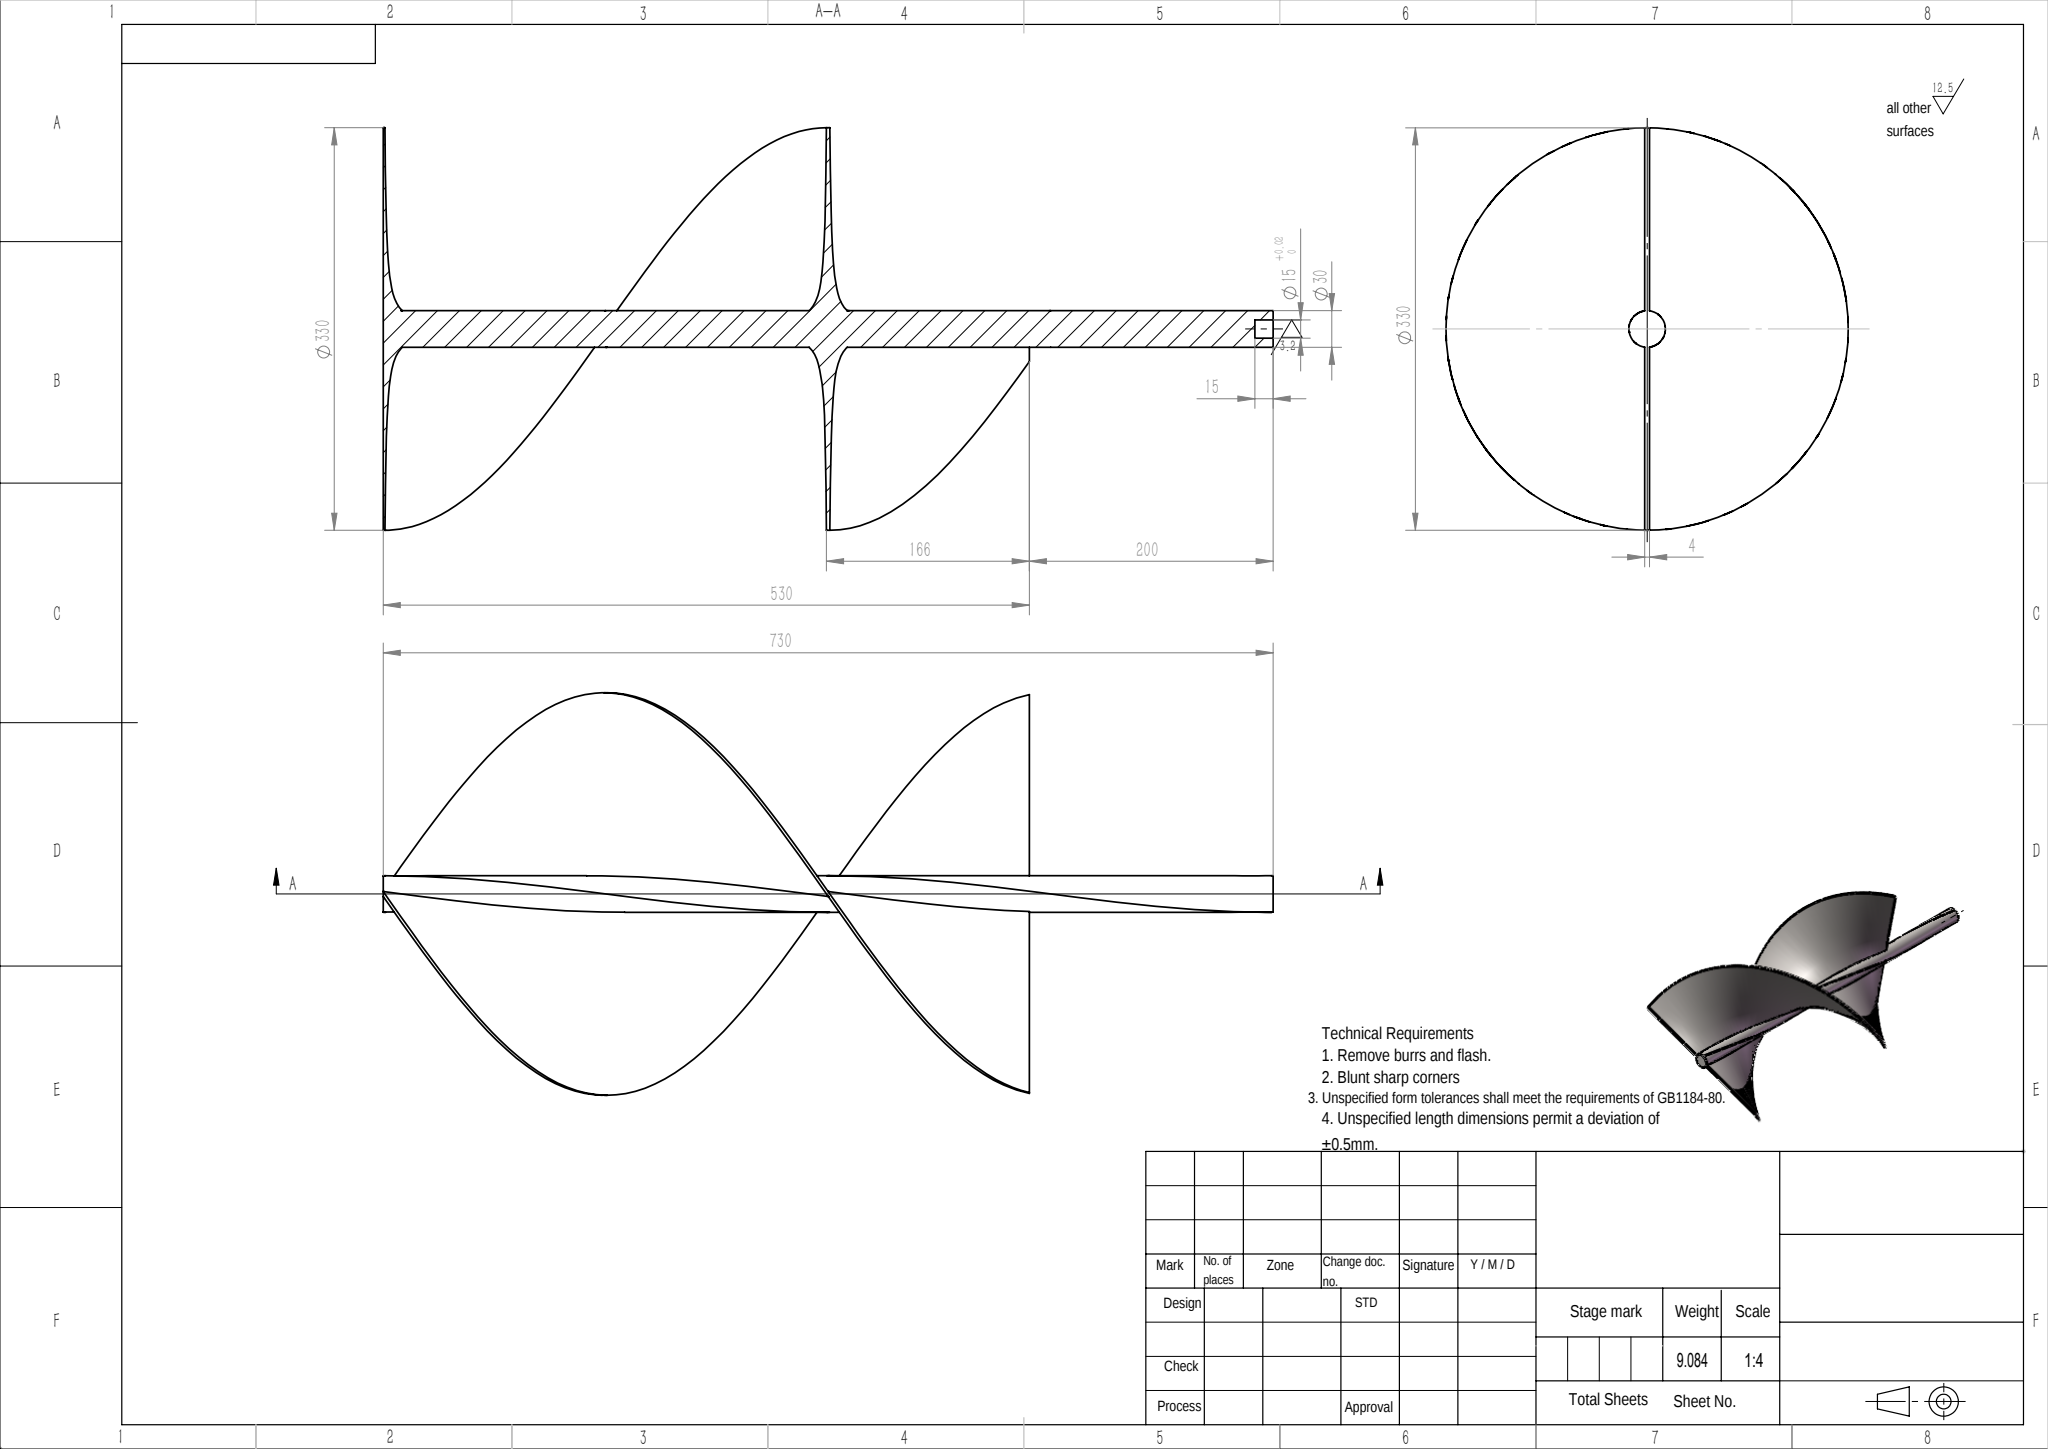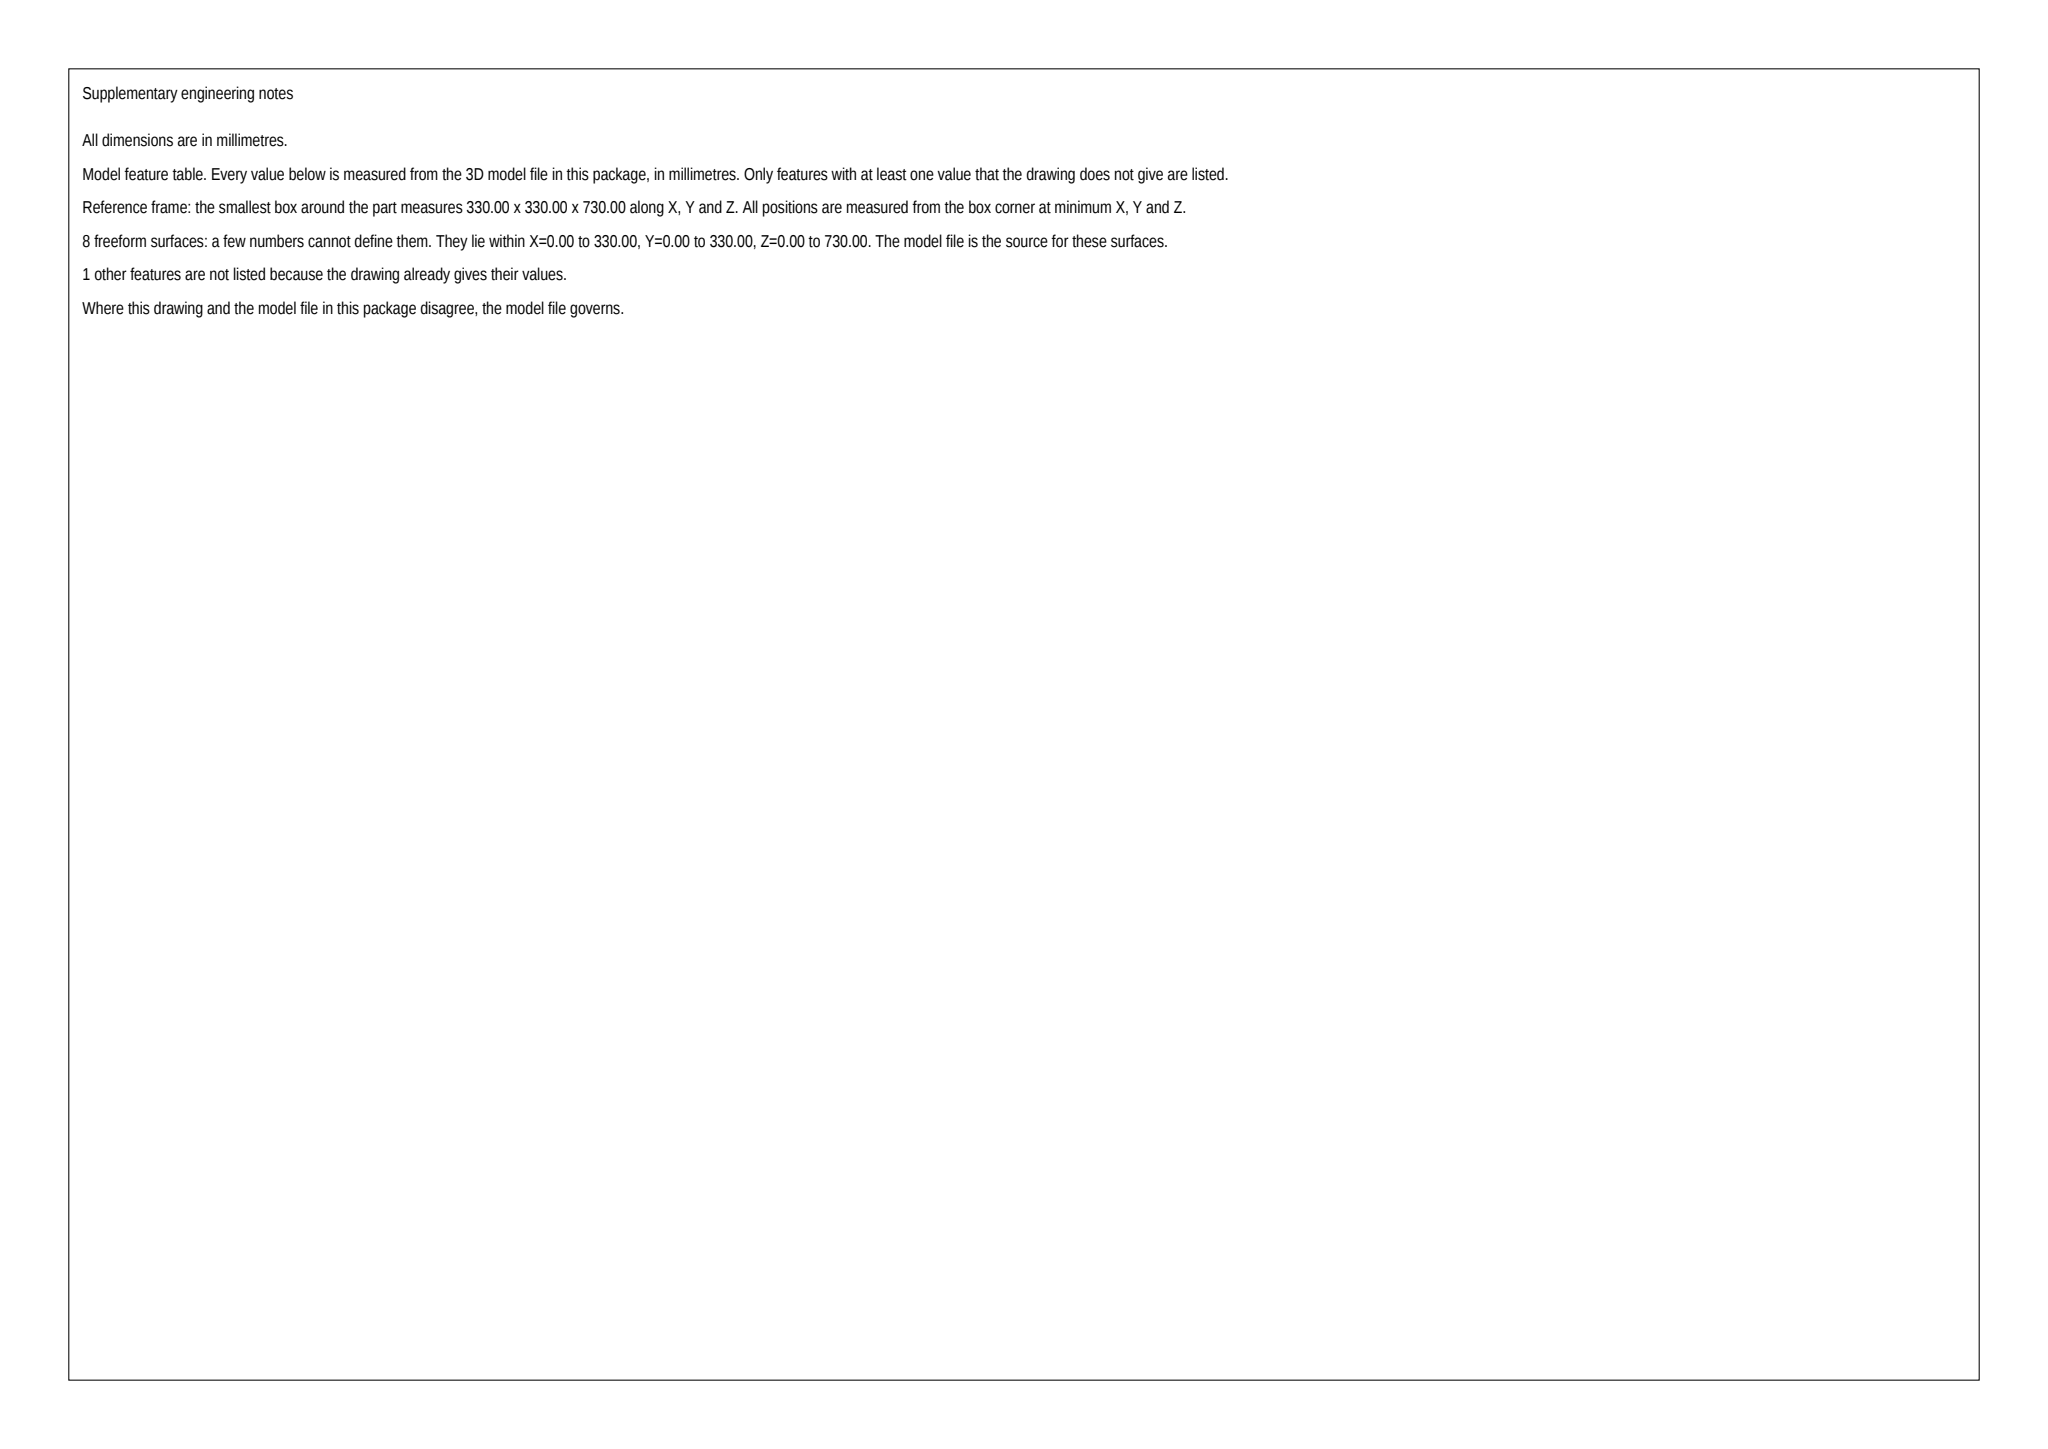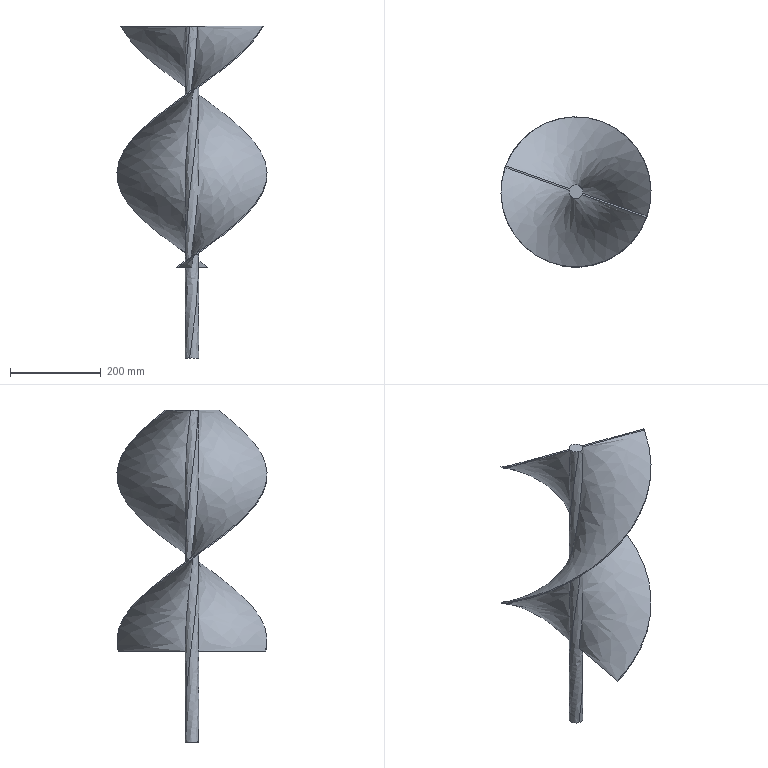Part | SolidWorks | mm | 1 solid | 15 faces | box 330 x 330 x 730 mm | volume 1149750 mm3 | spline 8 | plane 5 | cylinder 2 | commonest cylinder face diameters 15 x2
Drawing notes:
FLIGHT ZONE: 200 TO 730 FROM Ø15 END FACE, 530 TOTAL LG | from the solid: Planes z=0/15 (Ø15x15 journal), flight face z=200, bbox z=730.006
FLIGHT 1 (SHORT): 200 TO 366 FROM Ø15 END FACE, 166 LG, 1 FULL TURN, LEAD 166 | from the solid: Flight end planes z=200 (count 2); 166 step -> 200+166=366, 166 axial = 360 deg
FLIGHT 2 (LONG): 366 TO 730 FROM Ø15 END FACE, 364 LG, 1 FULL TURN, LEAD 364 | from the solid: Run from z=366 to end plane z=730.006; 530-166=364 axial = 360 deg